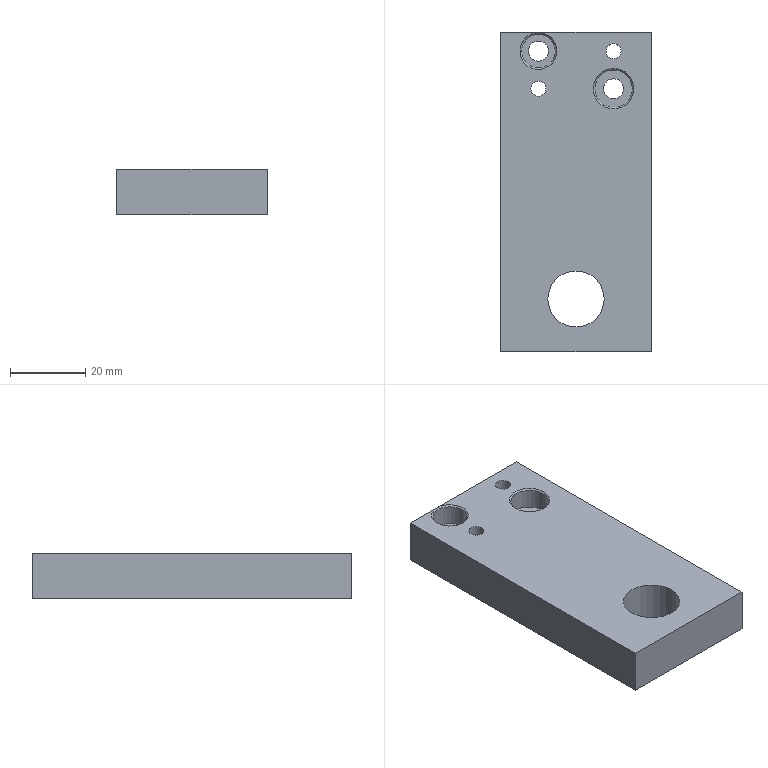Component | NX | DRILL_JIG | 1 solid | 19 faces | volume 37272 mm3 | plane 8 | cylinder 7 | cone 4 | commonest cylinder face diameters 5.3 x2 4 x2 15 x1 10 x1 9 x1